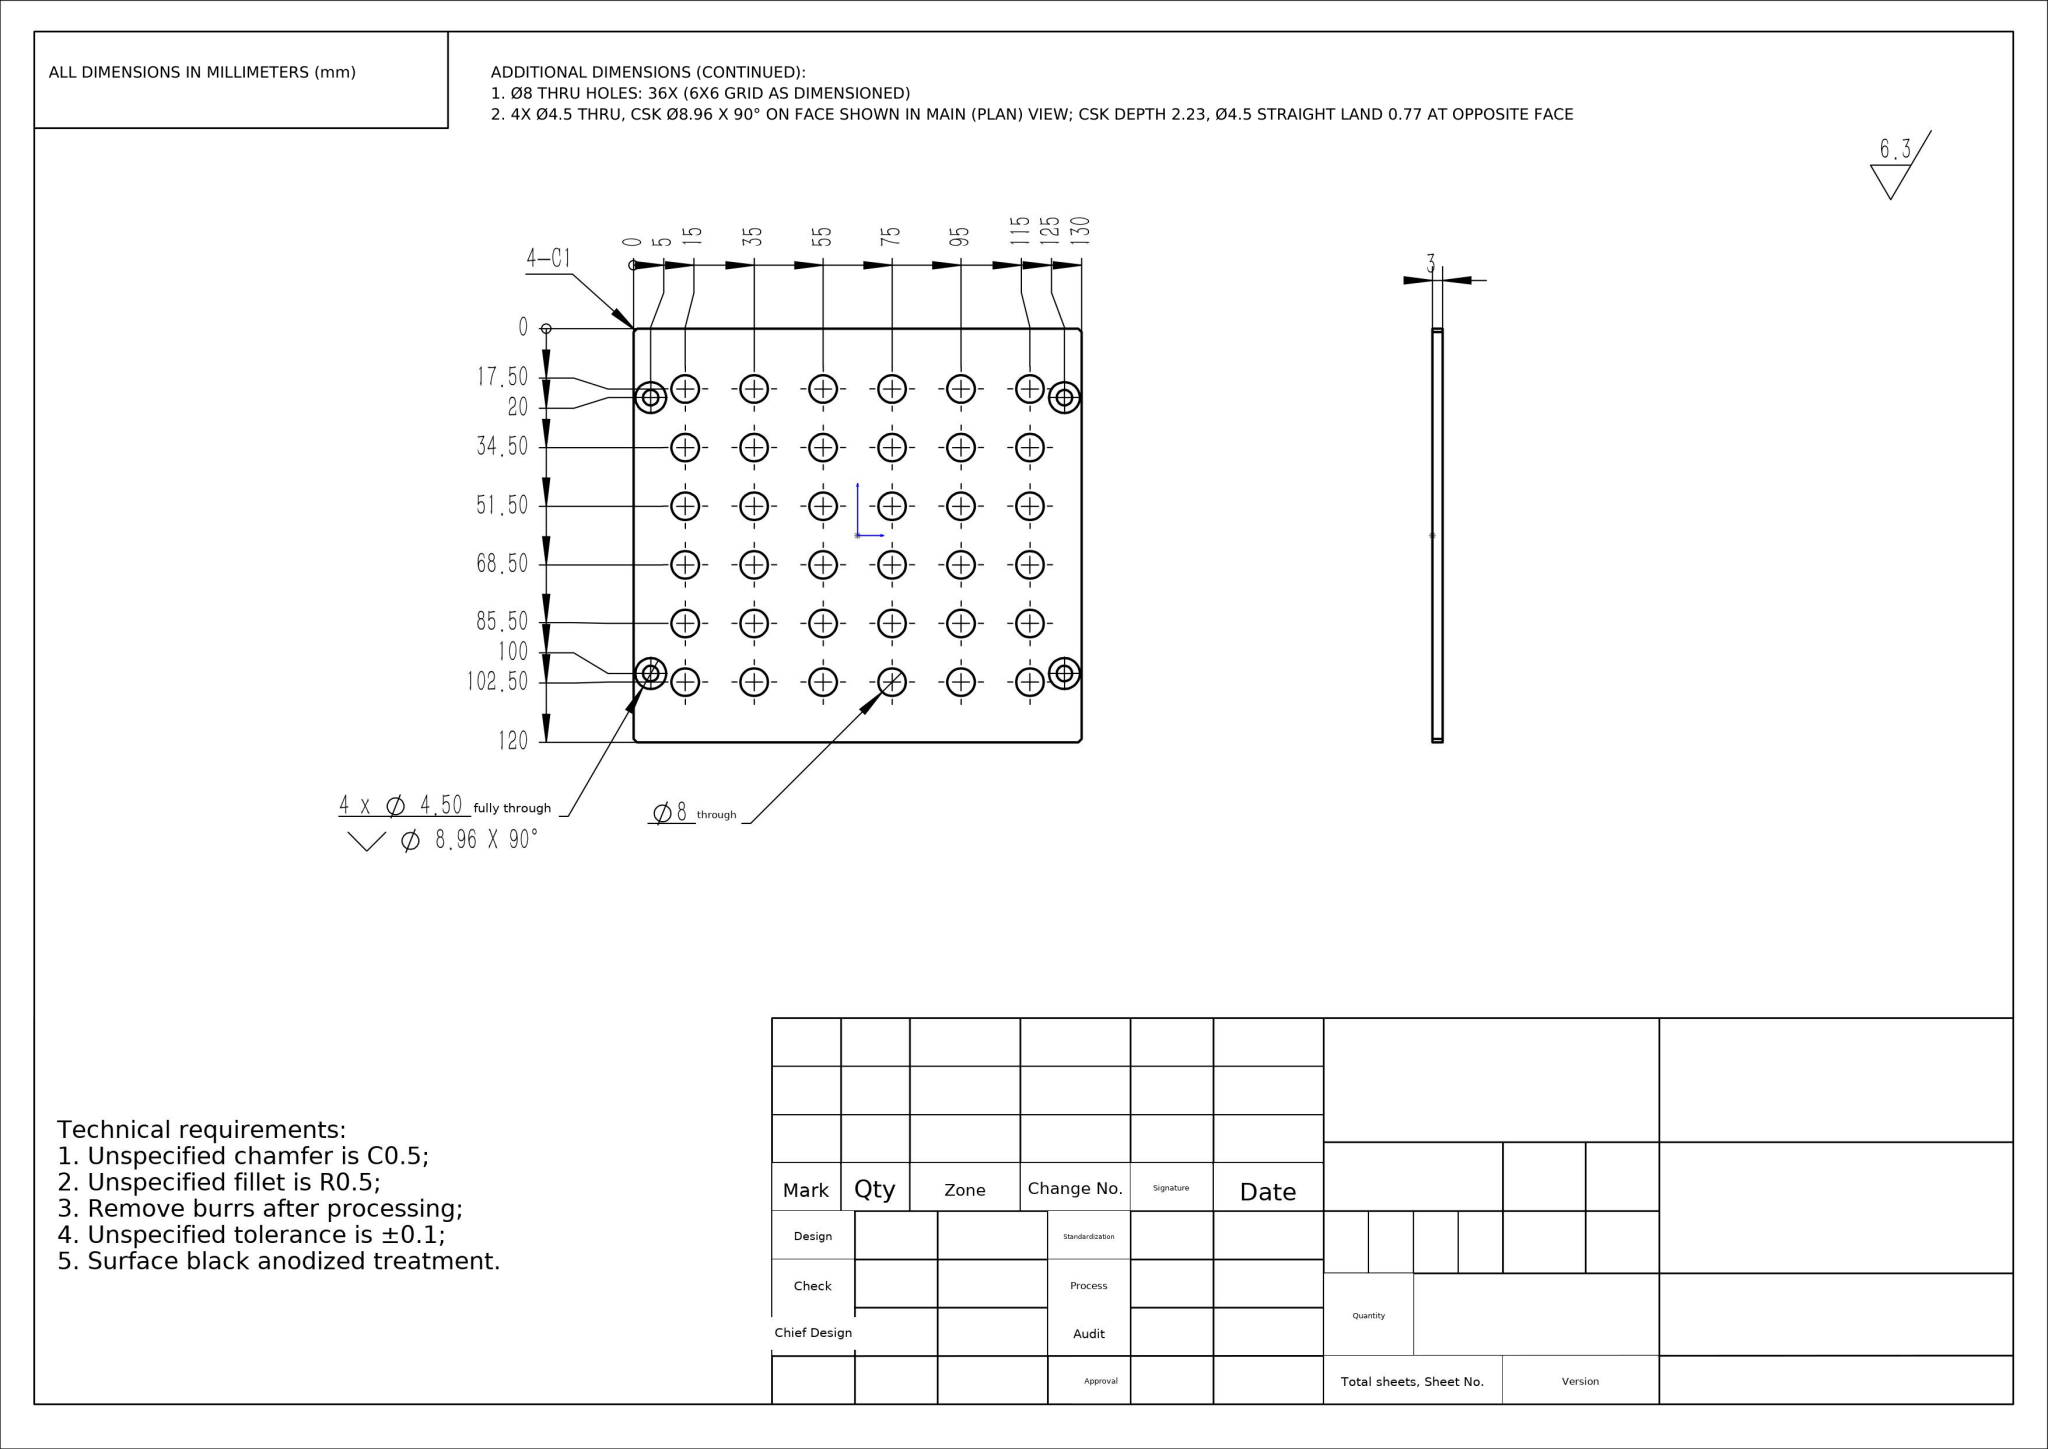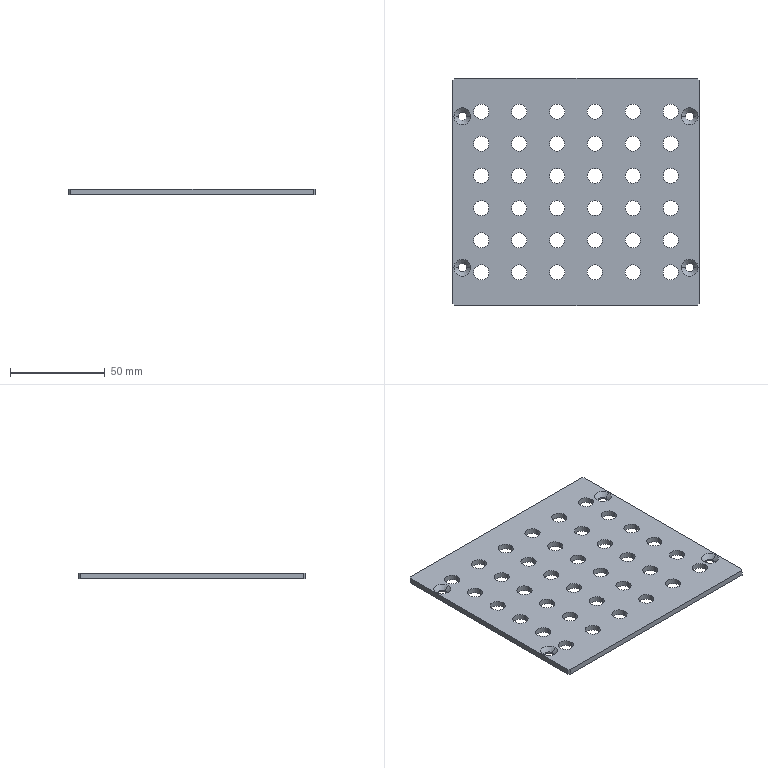Part | NX | mm | 1 solid | 98 faces | box 130 x 120 x 3 mm | volume 40987 mm3 | cylinder 80 | plane 10 | cone 8 | commonest cylinder face diameters 8 x72 4.5 x8